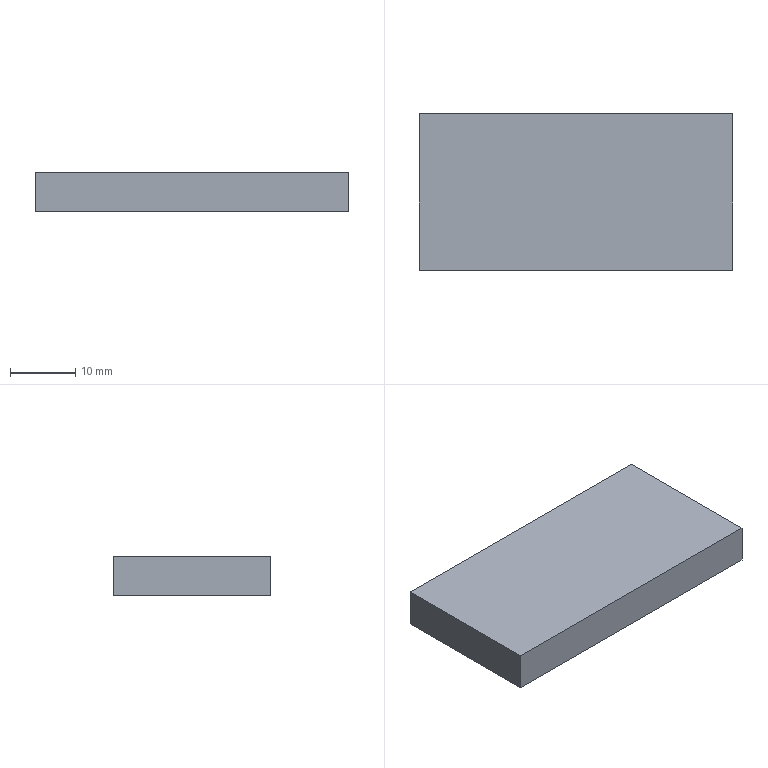Component | NX | TRANSFER_SURFACE | 1 solid | 6 faces | box 48 x 24 x 6 mm | volume 6912 mm3 | plane 6
STEP:
#1=CARTESIAN_POINT('',(0.,0.,0.));
#2=DIRECTION('',(0.,0.,1.));
#3=DIRECTION('',(1.,0.,0.));
#4=AXIS2_PLACEMENT_3D('',#1,#2,#3);
#5=CARTESIAN_POINT('',(28.064,-39.,12.));
#6=VERTEX_POINT('',#5);
#7=CARTESIAN_POINT('',(-19.936,-39.,12.));
#8=VERTEX_POINT('',#7);
#9=CARTESIAN_POINT('',(4.064,-39.,12.));
#10=DIRECTION('',(-1.,0.,0.));
#11=VECTOR('',#10,1.);
#12=LINE('',#9,#11);
#13=CARTESIAN_POINT('',(4.064,-27.,12.));
#14=DIRECTION('',(0.,0.,1.));
#15=DIRECTION('',(1.,0.,0.));
#16=AXIS2_PLACEMENT_3D('',#13,#14,#15);
#17=PLANE('',#16);
#18=CARTESIAN_POINT('',(0.,-12.));
#19=DIRECTION('',(-1.,0.));
#20=VECTOR('',#19,1.);
#21=LINE('',#18,#20);
#22=(GEOMETRIC_REPRESENTATION_CONTEXT(2)PARAMETRIC_REPRESENTATION_CONTEXT()REPRESENTATION_CONTEXT('',''));
#23=DEFINITIONAL_REPRESENTATION('',(#21),#22);
#24=PCURVE('',#17,#23);
#25=CARTESIAN_POINT('',(4.064,-39.,6.));
#26=DIRECTION('',(0.,-1.,0.));
#27=DIRECTION('',(0.,0.,-1.));
#28=AXIS2_PLACEMENT_3D('',#25,#26,#27);
#29=PLANE('',#28);
#30=CARTESIAN_POINT('',(-6.,0.));
#31=DIRECTION('',(0.,-1.));
#32=VECTOR('',#31,1.);
#33=LINE('',#30,#32);
#34=(GEOMETRIC_REPRESENTATION_CONTEXT(2)PARAMETRIC_REPRESENTATION_CONTEXT()REPRESENTATION_CONTEXT('',''));
#35=DEFINITIONAL_REPRESENTATION('',(#33),#34);
#36=PCURVE('',#29,#35);
#37=SURFACE_CURVE('',#12,(#24,#36),.PCURVE_S1.);
#38=EDGE_CURVE('',#6,#8,#37,.T.);
#39=ORIENTED_EDGE('',*,*,#38,.F.);
#40=CARTESIAN_POINT('',(28.064,-15.,12.));
#41=VERTEX_POINT('',#40);
#42=CARTESIAN_POINT('',(28.064,-27.,12.));
#43=DIRECTION('',(0.,-1.,0.));
#44=VECTOR('',#43,1.);
#45=LINE('',#42,#44);
#46=CARTESIAN_POINT('',(24.,0.));
#47=DIRECTION('',(0.,-1.));
#48=VECTOR('',#47,1.);
#49=LINE('',#46,#48);
#50=(GEOMETRIC_REPRESENTATION_CONTEXT(2)PARAMETRIC_REPRESENTATION_CONTEXT()REPRESENTATION_CONTEXT('',''));
#51=DEFINITIONAL_REPRESENTATION('',(#49),#50);
#52=PCURVE('',#17,#51);
#53=CARTESIAN_POINT('',(28.064,-27.,6.));
#54=DIRECTION('',(1.,0.,0.));
#55=DIRECTION('',(0.,0.,-1.));
#56=AXIS2_PLACEMENT_3D('',#53,#54,#55);
#57=PLANE('',#56);
#58=CARTESIAN_POINT('',(-6.,0.));
#59=DIRECTION('',(0.,-1.));
#60=VECTOR('',#59,1.);
#61=LINE('',#58,#60);
#62=(GEOMETRIC_REPRESENTATION_CONTEXT(2)PARAMETRIC_REPRESENTATION_CONTEXT()REPRESENTATION_CONTEXT('',''));
#63=DEFINITIONAL_REPRESENTATION('',(#61),#62);
#64=PCURVE('',#57,#63);
#65=SURFACE_CURVE('',#45,(#52,#64),.PCURVE_S1.);
#66=EDGE_CURVE('',#41,#6,#65,.T.);
#67=ORIENTED_EDGE('',*,*,#66,.F.);
#68=CARTESIAN_POINT('',(-19.936,-15.,12.));
#69=VERTEX_POINT('',#68);
#70=CARTESIAN_POINT('',(4.064,-15.,12.));
#71=DIRECTION('',(1.,0.,0.));
#72=VECTOR('',#71,1.);
#73=LINE('',#70,#72);
#74=CARTESIAN_POINT('',(0.,12.));
#75=DIRECTION('',(1.,0.));
#76=VECTOR('',#75,1.);
#77=LINE('',#74,#76);
#78=(GEOMETRIC_REPRESENTATION_CONTEXT(2)PARAMETRIC_REPRESENTATION_CONTEXT()REPRESENTATION_CONTEXT('',''));
#79=DEFINITIONAL_REPRESENTATION('',(#77),#78);
#80=PCURVE('',#17,#79);
#81=CARTESIAN_POINT('',(4.064,-15.,6.));
#82=DIRECTION('',(0.,1.,0.));
#83=DIRECTION('',(0.,0.,1.));
#84=AXIS2_PLACEMENT_3D('',#81,#82,#83);
#85=PLANE('',#84);
#86=CARTESIAN_POINT('',(6.,0.));
#87=DIRECTION('',(0.,1.));
#88=VECTOR('',#87,1.);
#89=LINE('',#86,#88);
#90=(GEOMETRIC_REPRESENTATION_CONTEXT(2)PARAMETRIC_REPRESENTATION_CONTEXT()REPRESENTATION_CONTEXT('',''));
#91=DEFINITIONAL_REPRESENTATION('',(#89),#90);
#92=PCURVE('',#85,#91);
#93=SURFACE_CURVE('',#73,(#80,#92),.PCURVE_S1.);
#94=EDGE_CURVE('',#69,#41,#93,.T.);
#95=ORIENTED_EDGE('',*,*,#94,.F.);
#96=CARTESIAN_POINT('',(-19.936,-27.,12.));
#97=DIRECTION('',(0.,1.,0.));
#98=VECTOR('',#97,1.);
#99=LINE('',#96,#98);
#100=CARTESIAN_POINT('',(-24.,0.));
#101=DIRECTION('',(0.,1.));
#102=VECTOR('',#101,1.);
#103=LINE('',#100,#102);
#104=(GEOMETRIC_REPRESENTATION_CONTEXT(2)PARAMETRIC_REPRESENTATION_CONTEXT()REPRESENTATION_CONTEXT('',''));
#105=DEFINITIONAL_REPRESENTATION('',(#103),#104);
#106=PCURVE('',#17,#105);
#107=CARTESIAN_POINT('',(-19.936,-27.,6.));
#108=DIRECTION('',(-1.,0.,0.));
#109=DIRECTION('',(0.,0.,1.));
#110=AXIS2_PLACEMENT_3D('',#107,#108,#109);
#111=PLANE('',#110);
#112=CARTESIAN_POINT('',(6.,0.));
#113=DIRECTION('',(0.,1.));
#114=VECTOR('',#113,1.);
#115=LINE('',#112,#114);
#116=(GEOMETRIC_REPRESENTATION_CONTEXT(2)PARAMETRIC_REPRESENTATION_CONTEXT()REPRESENTATION_CONTEXT('',''));
#117=DEFINITIONAL_REPRESENTATION('',(#115),#116);
#118=PCURVE('',#111,#117);
#119=SURFACE_CURVE('',#99,(#106,#118),.PCURVE_S1.);
#120=EDGE_CURVE('',#8,#69,#119,.T.);
#121=ORIENTED_EDGE('',*,*,#120,.F.);
#122=EDGE_LOOP('',(#39,#67,#95,#121));
#123=FACE_BOUND('',#122,.T.);
#124=ADVANCED_FACE('',(#123),#17,.T.);
#125=CARTESIAN_POINT('',(28.064,-39.,6.));
#126=VERTEX_POINT('',#125);
#127=CARTESIAN_POINT('',(28.064,-39.,6.));
#128=DIRECTION('',(0.,0.,1.));
#129=VECTOR('',#128,1.);
#130=LINE('',#127,#129);
#131=CARTESIAN_POINT('',(0.,24.));
#132=DIRECTION('',(-1.,0.));
#133=VECTOR('',#132,1.);
#134=LINE('',#131,#133);
#135=(GEOMETRIC_REPRESENTATION_CONTEXT(2)PARAMETRIC_REPRESENTATION_CONTEXT()REPRESENTATION_CONTEXT('',''));
#136=DEFINITIONAL_REPRESENTATION('',(#134),#135);
#137=PCURVE('',#29,#136);
#138=CARTESIAN_POINT('',(0.,-12.));
#139=DIRECTION('',(-1.,0.));
#140=VECTOR('',#139,1.);
#141=LINE('',#138,#140);
#142=(GEOMETRIC_REPRESENTATION_CONTEXT(2)PARAMETRIC_REPRESENTATION_CONTEXT()REPRESENTATION_CONTEXT('',''));
#143=DEFINITIONAL_REPRESENTATION('',(#141),#142);
#144=PCURVE('',#57,#143);
#145=SURFACE_CURVE('',#130,(#137,#144),.PCURVE_S1.);
#146=EDGE_CURVE('',#126,#6,#145,.T.);
#147=ORIENTED_EDGE('',*,*,#146,.T.);
#148=ORIENTED_EDGE('',*,*,#38,.T.);
#149=CARTESIAN_POINT('',(-19.936,-39.,6.));
#150=VERTEX_POINT('',#149);
#151=CARTESIAN_POINT('',(-19.936,-39.,6.));
#152=DIRECTION('',(0.,0.,1.));
#153=VECTOR('',#152,1.);
#154=LINE('',#151,#153);
#155=CARTESIAN_POINT('',(0.,-24.));
#156=DIRECTION('',(-1.,0.));
#157=VECTOR('',#156,1.);
#158=LINE('',#155,#157);
#159=(GEOMETRIC_REPRESENTATION_CONTEXT(2)PARAMETRIC_REPRESENTATION_CONTEXT()REPRESENTATION_CONTEXT('',''));
#160=DEFINITIONAL_REPRESENTATION('',(#158),#159);
#161=PCURVE('',#29,#160);
#162=CARTESIAN_POINT('',(0.,-12.));
#163=DIRECTION('',(1.,0.));
#164=VECTOR('',#163,1.);
#165=LINE('',#162,#164);
#166=(GEOMETRIC_REPRESENTATION_CONTEXT(2)PARAMETRIC_REPRESENTATION_CONTEXT()REPRESENTATION_CONTEXT('',''));
#167=DEFINITIONAL_REPRESENTATION('',(#165),#166);
#168=PCURVE('',#111,#167);
#169=SURFACE_CURVE('',#154,(#161,#168),.PCURVE_S1.);
#170=EDGE_CURVE('',#150,#8,#169,.T.);
#171=ORIENTED_EDGE('',*,*,#170,.F.);
#172=CARTESIAN_POINT('',(4.064,-39.,6.));
#173=DIRECTION('',(1.,0.,0.));
#174=VECTOR('',#173,1.);
#175=LINE('',#172,#174);
#176=CARTESIAN_POINT('',(0.,0.));
#177=DIRECTION('',(0.,1.));
#178=VECTOR('',#177,1.);
#179=LINE('',#176,#178);
#180=(GEOMETRIC_REPRESENTATION_CONTEXT(2)PARAMETRIC_REPRESENTATION_CONTEXT()REPRESENTATION_CONTEXT('',''));
#181=DEFINITIONAL_REPRESENTATION('',(#179),#180);
#182=PCURVE('',#29,#181);
#183=CARTESIAN_POINT('',(4.064,-27.,6.));
#184=DIRECTION('',(0.,0.,-1.));
#185=DIRECTION('',(-1.,0.,0.));
#186=AXIS2_PLACEMENT_3D('',#183,#184,#185);
#187=PLANE('',#186);
#188=CARTESIAN_POINT('',(0.,-12.));
#189=DIRECTION('',(-1.,0.));
#190=VECTOR('',#189,1.);
#191=LINE('',#188,#190);
#192=(GEOMETRIC_REPRESENTATION_CONTEXT(2)PARAMETRIC_REPRESENTATION_CONTEXT()REPRESENTATION_CONTEXT('',''));
#193=DEFINITIONAL_REPRESENTATION('',(#191),#192);
#194=PCURVE('',#187,#193);
#195=SURFACE_CURVE('',#175,(#182,#194),.PCURVE_S1.);
#196=EDGE_CURVE('',#150,#126,#195,.T.);
#197=ORIENTED_EDGE('',*,*,#196,.T.);
#198=EDGE_LOOP('',(#147,#148,#171,#197));
#199=FACE_BOUND('',#198,.T.);
#200=ADVANCED_FACE('',(#199),#29,.T.);
#201=ORIENTED_EDGE('',*,*,#170,.T.);
#202=ORIENTED_EDGE('',*,*,#120,.T.);
#203=CARTESIAN_POINT('',(-19.936,-15.,6.));
#204=VERTEX_POINT('',#203);
#205=CARTESIAN_POINT('',(-19.936,-15.,6.));
#206=DIRECTION('',(0.,0.,1.));
#207=VECTOR('',#206,1.);
#208=LINE('',#205,#207);
#209=CARTESIAN_POINT('',(0.,12.));
#210=DIRECTION('',(1.,0.));
#211=VECTOR('',#210,1.);
#212=LINE('',#209,#211);
#213=(GEOMETRIC_REPRESENTATION_CONTEXT(2)PARAMETRIC_REPRESENTATION_CONTEXT()REPRESENTATION_CONTEXT('',''));
#214=DEFINITIONAL_REPRESENTATION('',(#212),#213);
#215=PCURVE('',#111,#214);
#216=CARTESIAN_POINT('',(0.,-24.));
#217=DIRECTION('',(1.,0.));
#218=VECTOR('',#217,1.);
#219=LINE('',#216,#218);
#220=(GEOMETRIC_REPRESENTATION_CONTEXT(2)PARAMETRIC_REPRESENTATION_CONTEXT()REPRESENTATION_CONTEXT('',''));
#221=DEFINITIONAL_REPRESENTATION('',(#219),#220);
#222=PCURVE('',#85,#221);
#223=SURFACE_CURVE('',#208,(#215,#222),.PCURVE_S1.);
#224=EDGE_CURVE('',#204,#69,#223,.T.);
#225=ORIENTED_EDGE('',*,*,#224,.F.);
#226=CARTESIAN_POINT('',(-19.936,-27.,6.));
#227=DIRECTION('',(0.,-1.,0.));
#228=VECTOR('',#227,1.);
#229=LINE('',#226,#228);
#230=CARTESIAN_POINT('',(0.,0.));
#231=DIRECTION('',(0.,-1.));
#232=VECTOR('',#231,1.);
#233=LINE('',#230,#232);
#234=(GEOMETRIC_REPRESENTATION_CONTEXT(2)PARAMETRIC_REPRESENTATION_CONTEXT()REPRESENTATION_CONTEXT('',''));
#235=DEFINITIONAL_REPRESENTATION('',(#233),#234);
#236=PCURVE('',#111,#235);
#237=CARTESIAN_POINT('',(24.,0.));
#238=DIRECTION('',(0.,-1.));
#239=VECTOR('',#238,1.);
#240=LINE('',#237,#239);
#241=(GEOMETRIC_REPRESENTATION_CONTEXT(2)PARAMETRIC_REPRESENTATION_CONTEXT()REPRESENTATION_CONTEXT('',''));
#242=DEFINITIONAL_REPRESENTATION('',(#240),#241);
#243=PCURVE('',#187,#242);
#244=SURFACE_CURVE('',#229,(#236,#243),.PCURVE_S1.);
#245=EDGE_CURVE('',#204,#150,#244,.T.);
#246=ORIENTED_EDGE('',*,*,#245,.T.);
#247=EDGE_LOOP('',(#201,#202,#225,#246));
#248=FACE_BOUND('',#247,.T.);
#249=ADVANCED_FACE('',(#248),#111,.T.);
#250=ORIENTED_EDGE('',*,*,#224,.T.);
#251=ORIENTED_EDGE('',*,*,#94,.T.);
#252=CARTESIAN_POINT('',(28.064,-15.,6.));
#253=VERTEX_POINT('',#252);
#254=CARTESIAN_POINT('',(28.064,-15.,6.));
#255=DIRECTION('',(0.,0.,1.));
#256=VECTOR('',#255,1.);
#257=LINE('',#254,#256);
#258=CARTESIAN_POINT('',(0.,24.));
#259=DIRECTION('',(1.,0.));
#260=VECTOR('',#259,1.);
#261=LINE('',#258,#260);
#262=(GEOMETRIC_REPRESENTATION_CONTEXT(2)PARAMETRIC_REPRESENTATION_CONTEXT()REPRESENTATION_CONTEXT('',''));
#263=DEFINITIONAL_REPRESENTATION('',(#261),#262);
#264=PCURVE('',#85,#263);
#265=CARTESIAN_POINT('',(0.,12.));
#266=DIRECTION('',(-1.,0.));
#267=VECTOR('',#266,1.);
#268=LINE('',#265,#267);
#269=(GEOMETRIC_REPRESENTATION_CONTEXT(2)PARAMETRIC_REPRESENTATION_CONTEXT()REPRESENTATION_CONTEXT('',''));
#270=DEFINITIONAL_REPRESENTATION('',(#268),#269);
#271=PCURVE('',#57,#270);
#272=SURFACE_CURVE('',#257,(#264,#271),.PCURVE_S1.);
#273=EDGE_CURVE('',#253,#41,#272,.T.);
#274=ORIENTED_EDGE('',*,*,#273,.F.);
#275=CARTESIAN_POINT('',(4.064,-15.,6.));
#276=DIRECTION('',(-1.,0.,0.));
#277=VECTOR('',#276,1.);
#278=LINE('',#275,#277);
#279=CARTESIAN_POINT('',(0.,0.));
#280=DIRECTION('',(0.,-1.));
#281=VECTOR('',#280,1.);
#282=LINE('',#279,#281);
#283=(GEOMETRIC_REPRESENTATION_CONTEXT(2)PARAMETRIC_REPRESENTATION_CONTEXT()REPRESENTATION_CONTEXT('',''));
#284=DEFINITIONAL_REPRESENTATION('',(#282),#283);
#285=PCURVE('',#85,#284);
#286=CARTESIAN_POINT('',(0.,12.));
#287=DIRECTION('',(1.,0.));
#288=VECTOR('',#287,1.);
#289=LINE('',#286,#288);
#290=(GEOMETRIC_REPRESENTATION_CONTEXT(2)PARAMETRIC_REPRESENTATION_CONTEXT()REPRESENTATION_CONTEXT('',''));
#291=DEFINITIONAL_REPRESENTATION('',(#289),#290);
#292=PCURVE('',#187,#291);
#293=SURFACE_CURVE('',#278,(#285,#292),.PCURVE_S1.);
#294=EDGE_CURVE('',#253,#204,#293,.T.);
#295=ORIENTED_EDGE('',*,*,#294,.T.);
#296=EDGE_LOOP('',(#250,#251,#274,#295));
#297=FACE_BOUND('',#296,.T.);
#298=ADVANCED_FACE('',(#297),#85,.T.);
#299=CARTESIAN_POINT('',(28.064,-27.,6.));
#300=DIRECTION('',(0.,1.,0.));
#301=VECTOR('',#300,1.);
#302=LINE('',#299,#301);
#303=CARTESIAN_POINT('',(-24.,0.));
#304=DIRECTION('',(0.,1.));
#305=VECTOR('',#304,1.);
#306=LINE('',#303,#305);
#307=(GEOMETRIC_REPRESENTATION_CONTEXT(2)PARAMETRIC_REPRESENTATION_CONTEXT()REPRESENTATION_CONTEXT('',''));
#308=DEFINITIONAL_REPRESENTATION('',(#306),#307);
#309=PCURVE('',#187,#308);
#310=CARTESIAN_POINT('',(0.,0.));
#311=DIRECTION('',(0.,1.));
#312=VECTOR('',#311,1.);
#313=LINE('',#310,#312);
#314=(GEOMETRIC_REPRESENTATION_CONTEXT(2)PARAMETRIC_REPRESENTATION_CONTEXT()REPRESENTATION_CONTEXT('',''));
#315=DEFINITIONAL_REPRESENTATION('',(#313),#314);
#316=PCURVE('',#57,#315);
#317=SURFACE_CURVE('',#302,(#309,#316),.PCURVE_S1.);
#318=EDGE_CURVE('',#126,#253,#317,.T.);
#319=ORIENTED_EDGE('',*,*,#318,.F.);
#320=ORIENTED_EDGE('',*,*,#196,.F.);
#321=ORIENTED_EDGE('',*,*,#245,.F.);
#322=ORIENTED_EDGE('',*,*,#294,.F.);
#323=EDGE_LOOP('',(#319,#320,#321,#322));
#324=FACE_BOUND('',#323,.T.);
#325=ADVANCED_FACE('',(#324),#187,.T.);
#326=ORIENTED_EDGE('',*,*,#318,.T.);
#327=ORIENTED_EDGE('',*,*,#273,.T.);
#328=ORIENTED_EDGE('',*,*,#66,.T.);
#329=ORIENTED_EDGE('',*,*,#146,.F.);
#330=EDGE_LOOP('',(#326,#327,#328,#329));
#331=FACE_BOUND('',#330,.T.);
#332=ADVANCED_FACE('',(#331),#57,.T.);
#333=CLOSED_SHELL('',(#124,#200,#249,#298,#325,#332));
#334=MANIFOLD_SOLID_BREP('',#333);
#335=(LENGTH_UNIT()NAMED_UNIT(*)SI_UNIT(.MILLI.,.METRE.));
#336=UNCERTAINTY_MEASURE_WITH_UNIT(LENGTH_MEASURE(0.0000001),#335,'','');
#337=(NAMED_UNIT(*)PLANE_ANGLE_UNIT()SI_UNIT($,.RADIAN.));
#338=(NAMED_UNIT(*)SI_UNIT($,.STERADIAN.)SOLID_ANGLE_UNIT());
#339=(GEOMETRIC_REPRESENTATION_CONTEXT(3)GLOBAL_UNCERTAINTY_ASSIGNED_CONTEXT((#336))GLOBAL_UNIT_ASSIGNED_CONTEXT((#335,#337,#338))REPRESENTATION_CONTEXT('',''));
#340=ADVANCED_BREP_SHAPE_REPRESENTATION('',(#4,#334),#339);